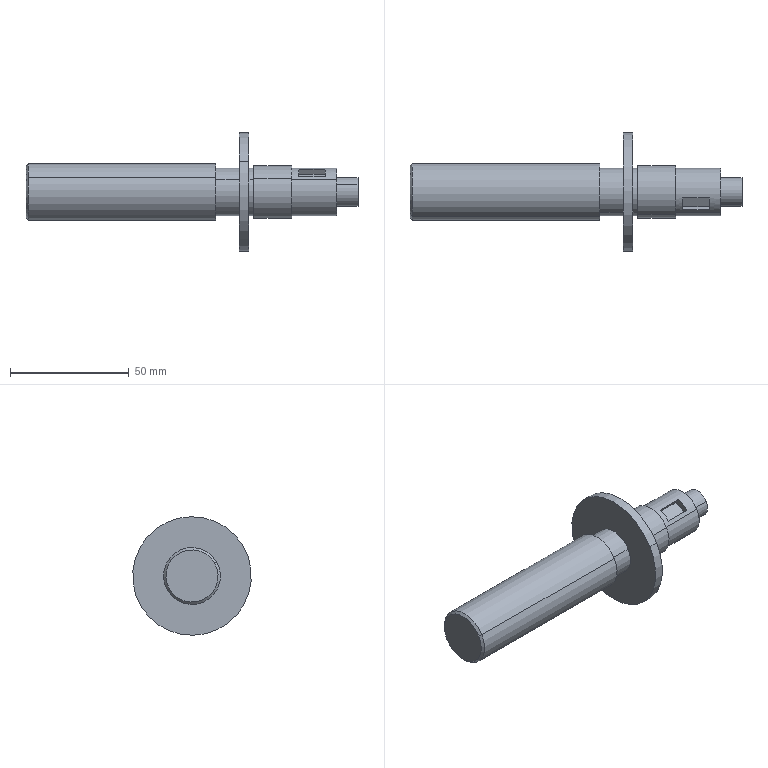Component | SolidWorks | ScrewRod-1 | 1 solid | 29 faces | box 140 x 50 x 50 mm | volume 60656 mm3 | cylinder 14 | plane 13 | cone 2 | commonest cylinder face diameters 20 x6 24 x2 50 x2 22 x2 12 x2
STEP:
#1=COLOUR_RGB('',0.7922,0.8196,0.9333);
#2=FILL_AREA_STYLE_COLOUR('',#1);
#3=FILL_AREA_STYLE('',(#2));
#4=SURFACE_STYLE_FILL_AREA(#3);
#5=SURFACE_SIDE_STYLE('',(#4));
#6=SURFACE_STYLE_USAGE(.BOTH.,#5);
#7=PRESENTATION_STYLE_ASSIGNMENT((#6));
#8=CARTESIAN_POINT('',(0.7305,6.278,-0.8121));
#9=VERTEX_POINT('',#8);
#10=CARTESIAN_POINT('',(0.7305,5.533,-0.369));
#11=VERTEX_POINT('',#10);
#12=CARTESIAN_POINT('',(0.7305,5.906,-0.5906));
#13=DIRECTION('',(-1.,-0.,0.));
#14=DIRECTION('',(0.,-0.8593,0.5115));
#15=AXIS2_PLACEMENT_3D('',#12,#13,#14);
#16=CIRCLE('',#15,0.4331);
#17=EDGE_CURVE('',#9,#11,#16,.T.);
#18=ORIENTED_EDGE('',*,*,#17,.F.);
#19=CARTESIAN_POINT('',(0.7699,6.311,-0.8322));
#20=VERTEX_POINT('',#19);
#21=CARTESIAN_POINT('',(0.7305,6.278,-0.8121));
#22=DIRECTION('',(0.7071,0.6076,-0.3617));
#23=VECTOR('',#22,39.37);
#24=LINE('',#21,#23);
#25=EDGE_CURVE('',#9,#20,#24,.T.);
#26=ORIENTED_EDGE('',*,*,#25,.T.);
#27=CARTESIAN_POINT('',(0.7699,5.5,-0.3489));
#28=VERTEX_POINT('',#27);
#29=CARTESIAN_POINT('',(0.7699,5.906,-0.5906));
#30=DIRECTION('',(1.,0.,-0.));
#31=DIRECTION('',(0.,-0.8593,0.5115));
#32=AXIS2_PLACEMENT_3D('',#29,#30,#31);
#33=CIRCLE('',#32,0.4724);
#34=EDGE_CURVE('',#28,#20,#33,.T.);
#35=ORIENTED_EDGE('',*,*,#34,.F.);
#36=CARTESIAN_POINT('',(0.7305,5.533,-0.369));
#37=DIRECTION('',(0.7071,-0.6076,0.3617));
#38=VECTOR('',#37,39.37);
#39=LINE('',#36,#38);
#40=EDGE_CURVE('',#11,#28,#39,.T.);
#41=ORIENTED_EDGE('',*,*,#40,.F.);
#42=EDGE_LOOP('',(#18,#26,#35,#41));
#43=FACE_OUTER_BOUND('',#42,.T.);
#44=CARTESIAN_POINT('',(0.7305,5.906,-0.5906));
#45=DIRECTION('',(1.,0.,-0.));
#46=DIRECTION('',(0.,-0.8593,0.5115));
#47=AXIS2_PLACEMENT_3D('',#44,#45,#46);
#48=CONICAL_SURFACE('',#47,0.4331,0.7854);
#49=ADVANCED_FACE('',(#43),#48,.T.);
#50=CARTESIAN_POINT('',(3.88,6.311,-0.8322));
#51=VERTEX_POINT('',#50);
#52=CARTESIAN_POINT('',(3.88,5.5,-0.3489));
#53=VERTEX_POINT('',#52);
#54=CARTESIAN_POINT('',(3.88,5.906,-0.5906));
#55=DIRECTION('',(-1.,-0.,0.));
#56=DIRECTION('',(0.,0.8593,-0.5115));
#57=AXIS2_PLACEMENT_3D('',#54,#55,#56);
#58=CIRCLE('',#57,0.4724);
#59=EDGE_CURVE('',#51,#53,#58,.T.);
#60=ORIENTED_EDGE('',*,*,#59,.T.);
#61=CARTESIAN_POINT('',(0.7305,5.5,-0.3489));
#62=DIRECTION('',(-1.,-0.,0.));
#63=VECTOR('',#62,39.37);
#64=LINE('',#61,#63);
#65=EDGE_CURVE('',#53,#28,#64,.T.);
#66=ORIENTED_EDGE('',*,*,#65,.T.);
#67=ORIENTED_EDGE('',*,*,#34,.T.);
#68=CARTESIAN_POINT('',(0.7305,6.311,-0.8322));
#69=DIRECTION('',(-1.,-0.,0.));
#70=VECTOR('',#69,39.37);
#71=LINE('',#68,#70);
#72=EDGE_CURVE('',#51,#20,#71,.T.);
#73=ORIENTED_EDGE('',*,*,#72,.F.);
#74=EDGE_LOOP('',(#60,#66,#67,#73));
#75=FACE_OUTER_BOUND('',#74,.T.);
#76=CARTESIAN_POINT('',(0.7305,5.906,-0.5906));
#77=DIRECTION('',(-1.,-0.,0.));
#78=DIRECTION('',(0.,0.8593,-0.5115));
#79=AXIS2_PLACEMENT_3D('',#76,#77,#78);
#80=CYLINDRICAL_SURFACE('',#79,0.4724);
#81=ADVANCED_FACE('',(#75),#80,.T.);
#82=CARTESIAN_POINT('',(4.274,6.244,-0.7919));
#83=VERTEX_POINT('',#82);
#84=CARTESIAN_POINT('',(4.274,5.567,-0.3892));
#85=VERTEX_POINT('',#84);
#86=CARTESIAN_POINT('',(4.274,5.906,-0.5906));
#87=DIRECTION('',(-1.,-0.,0.));
#88=DIRECTION('',(0.,0.8593,-0.5115));
#89=AXIS2_PLACEMENT_3D('',#86,#87,#88);
#90=CIRCLE('',#89,0.3937);
#91=EDGE_CURVE('',#83,#85,#90,.T.);
#92=ORIENTED_EDGE('',*,*,#91,.T.);
#93=CARTESIAN_POINT('',(3.88,5.567,-0.3892));
#94=VERTEX_POINT('',#93);
#95=CARTESIAN_POINT('',(0.7305,5.567,-0.3892));
#96=DIRECTION('',(-1.,-0.,0.));
#97=VECTOR('',#96,39.37);
#98=LINE('',#95,#97);
#99=EDGE_CURVE('',#85,#94,#98,.T.);
#100=ORIENTED_EDGE('',*,*,#99,.T.);
#101=CARTESIAN_POINT('',(3.88,6.244,-0.7919));
#102=VERTEX_POINT('',#101);
#103=CARTESIAN_POINT('',(3.88,5.906,-0.5906));
#104=DIRECTION('',(-1.,-0.,0.));
#105=DIRECTION('',(0.,0.8593,-0.5115));
#106=AXIS2_PLACEMENT_3D('',#103,#104,#105);
#107=CIRCLE('',#106,0.3937);
#108=EDGE_CURVE('',#102,#94,#107,.T.);
#109=ORIENTED_EDGE('',*,*,#108,.F.);
#110=CARTESIAN_POINT('',(0.7305,6.244,-0.7919));
#111=DIRECTION('',(-1.,-0.,0.));
#112=VECTOR('',#111,39.37);
#113=LINE('',#110,#112);
#114=EDGE_CURVE('',#83,#102,#113,.T.);
#115=ORIENTED_EDGE('',*,*,#114,.F.);
#116=EDGE_LOOP('',(#92,#100,#109,#115));
#117=FACE_OUTER_BOUND('',#116,.T.);
#118=CARTESIAN_POINT('',(0.7305,5.906,-0.5906));
#119=DIRECTION('',(-1.,-0.,0.));
#120=DIRECTION('',(0.,0.8593,-0.5115));
#121=AXIS2_PLACEMENT_3D('',#118,#119,#120);
#122=CYLINDRICAL_SURFACE('',#121,0.3937);
#123=ADVANCED_FACE('',(#117),#122,.T.);
#124=CARTESIAN_POINT('',(4.431,6.751,-1.094));
#125=VERTEX_POINT('',#124);
#126=CARTESIAN_POINT('',(4.431,5.06,-0.08708));
#127=VERTEX_POINT('',#126);
#128=CARTESIAN_POINT('',(4.431,5.906,-0.5906));
#129=DIRECTION('',(-1.,-0.,0.));
#130=DIRECTION('',(0.,0.8593,-0.5115));
#131=AXIS2_PLACEMENT_3D('',#128,#129,#130);
#132=CIRCLE('',#131,0.9843);
#133=EDGE_CURVE('',#125,#127,#132,.T.);
#134=ORIENTED_EDGE('',*,*,#133,.T.);
#135=CARTESIAN_POINT('',(4.274,5.06,-0.08708));
#136=VERTEX_POINT('',#135);
#137=CARTESIAN_POINT('',(0.7305,5.06,-0.08708));
#138=DIRECTION('',(-1.,-0.,0.));
#139=VECTOR('',#138,39.37);
#140=LINE('',#137,#139);
#141=EDGE_CURVE('',#127,#136,#140,.T.);
#142=ORIENTED_EDGE('',*,*,#141,.T.);
#143=CARTESIAN_POINT('',(4.274,6.751,-1.094));
#144=VERTEX_POINT('',#143);
#145=CARTESIAN_POINT('',(4.274,5.906,-0.5906));
#146=DIRECTION('',(-1.,-0.,0.));
#147=DIRECTION('',(0.,0.8593,-0.5115));
#148=AXIS2_PLACEMENT_3D('',#145,#146,#147);
#149=CIRCLE('',#148,0.9843);
#150=EDGE_CURVE('',#144,#136,#149,.T.);
#151=ORIENTED_EDGE('',*,*,#150,.F.);
#152=CARTESIAN_POINT('',(0.7305,6.751,-1.094));
#153=DIRECTION('',(-1.,-0.,0.));
#154=VECTOR('',#153,39.37);
#155=LINE('',#152,#154);
#156=EDGE_CURVE('',#125,#144,#155,.T.);
#157=ORIENTED_EDGE('',*,*,#156,.F.);
#158=EDGE_LOOP('',(#134,#142,#151,#157));
#159=FACE_OUTER_BOUND('',#158,.T.);
#160=CARTESIAN_POINT('',(0.7305,5.906,-0.5906));
#161=DIRECTION('',(-1.,-0.,0.));
#162=DIRECTION('',(-0.,0.8593,-0.5115));
#163=AXIS2_PLACEMENT_3D('',#160,#161,#162);
#164=CYLINDRICAL_SURFACE('',#163,0.9843);
#165=ADVANCED_FACE('',(#159),#164,.T.);
#166=CARTESIAN_POINT('',(4.51,6.244,-0.7919));
#167=VERTEX_POINT('',#166);
#168=CARTESIAN_POINT('',(4.51,5.567,-0.3892));
#169=VERTEX_POINT('',#168);
#170=CARTESIAN_POINT('',(4.51,5.906,-0.5906));
#171=DIRECTION('',(-1.,-0.,0.));
#172=DIRECTION('',(0.,0.8593,-0.5115));
#173=AXIS2_PLACEMENT_3D('',#170,#171,#172);
#174=CIRCLE('',#173,0.3937);
#175=EDGE_CURVE('',#167,#169,#174,.T.);
#176=ORIENTED_EDGE('',*,*,#175,.T.);
#177=CARTESIAN_POINT('',(4.431,5.567,-0.3892));
#178=VERTEX_POINT('',#177);
#179=CARTESIAN_POINT('',(0.7305,5.567,-0.3892));
#180=DIRECTION('',(-1.,-0.,0.));
#181=VECTOR('',#180,39.37);
#182=LINE('',#179,#181);
#183=EDGE_CURVE('',#169,#178,#182,.T.);
#184=ORIENTED_EDGE('',*,*,#183,.T.);
#185=CARTESIAN_POINT('',(4.431,6.244,-0.7919));
#186=VERTEX_POINT('',#185);
#187=CARTESIAN_POINT('',(4.431,5.906,-0.5906));
#188=DIRECTION('',(-1.,-0.,0.));
#189=DIRECTION('',(0.,0.8593,-0.5115));
#190=AXIS2_PLACEMENT_3D('',#187,#188,#189);
#191=CIRCLE('',#190,0.3937);
#192=EDGE_CURVE('',#186,#178,#191,.T.);
#193=ORIENTED_EDGE('',*,*,#192,.F.);
#194=CARTESIAN_POINT('',(0.7305,6.244,-0.7919));
#195=DIRECTION('',(-1.,-0.,0.));
#196=VECTOR('',#195,39.37);
#197=LINE('',#194,#196);
#198=EDGE_CURVE('',#167,#186,#197,.T.);
#199=ORIENTED_EDGE('',*,*,#198,.F.);
#200=EDGE_LOOP('',(#176,#184,#193,#199));
#201=FACE_OUTER_BOUND('',#200,.T.);
#202=CARTESIAN_POINT('',(0.7305,5.906,-0.5906));
#203=DIRECTION('',(-1.,-0.,0.));
#204=DIRECTION('',(0.,0.8593,-0.5115));
#205=AXIS2_PLACEMENT_3D('',#202,#203,#204);
#206=CYLINDRICAL_SURFACE('',#205,0.3937);
#207=ADVANCED_FACE('',(#201),#206,.T.);
#208=CARTESIAN_POINT('',(5.14,6.278,-0.8121));
#209=VERTEX_POINT('',#208);
#210=CARTESIAN_POINT('',(5.14,5.533,-0.369));
#211=VERTEX_POINT('',#210);
#212=CARTESIAN_POINT('',(5.14,5.906,-0.5906));
#213=DIRECTION('',(-1.,-0.,0.));
#214=DIRECTION('',(0.,0.8593,-0.5115));
#215=AXIS2_PLACEMENT_3D('',#212,#213,#214);
#216=CIRCLE('',#215,0.4331);
#217=EDGE_CURVE('',#209,#211,#216,.T.);
#218=ORIENTED_EDGE('',*,*,#217,.T.);
#219=CARTESIAN_POINT('',(4.51,5.533,-0.369));
#220=VERTEX_POINT('',#219);
#221=CARTESIAN_POINT('',(0.7305,5.533,-0.369));
#222=DIRECTION('',(-1.,-0.,0.));
#223=VECTOR('',#222,39.37);
#224=LINE('',#221,#223);
#225=EDGE_CURVE('',#211,#220,#224,.T.);
#226=ORIENTED_EDGE('',*,*,#225,.T.);
#227=CARTESIAN_POINT('',(4.51,6.278,-0.8121));
#228=VERTEX_POINT('',#227);
#229=CARTESIAN_POINT('',(4.51,5.906,-0.5906));
#230=DIRECTION('',(-1.,-0.,0.));
#231=DIRECTION('',(0.,0.8593,-0.5115));
#232=AXIS2_PLACEMENT_3D('',#229,#230,#231);
#233=CIRCLE('',#232,0.4331);
#234=EDGE_CURVE('',#228,#220,#233,.T.);
#235=ORIENTED_EDGE('',*,*,#234,.F.);
#236=CARTESIAN_POINT('',(0.7305,6.278,-0.8121));
#237=DIRECTION('',(-1.,-0.,0.));
#238=VECTOR('',#237,39.37);
#239=LINE('',#236,#238);
#240=EDGE_CURVE('',#209,#228,#239,.T.);
#241=ORIENTED_EDGE('',*,*,#240,.F.);
#242=EDGE_LOOP('',(#218,#226,#235,#241));
#243=FACE_OUTER_BOUND('',#242,.T.);
#244=CARTESIAN_POINT('',(0.7305,5.906,-0.5906));
#245=DIRECTION('',(-1.,-0.,0.));
#246=DIRECTION('',(0.,0.8593,-0.5115));
#247=AXIS2_PLACEMENT_3D('',#244,#245,#246);
#248=CYLINDRICAL_SURFACE('',#247,0.4331);
#249=ADVANCED_FACE('',(#243),#248,.T.);
#250=CARTESIAN_POINT('',(6.242,6.108,-0.7114));
#251=VERTEX_POINT('',#250);
#252=CARTESIAN_POINT('',(6.242,5.703,-0.4697));
#253=VERTEX_POINT('',#252);
#254=CARTESIAN_POINT('',(6.242,5.906,-0.5906));
#255=DIRECTION('',(-1.,-0.,0.));
#256=DIRECTION('',(0.,0.8593,-0.5115));
#257=AXIS2_PLACEMENT_3D('',#254,#255,#256);
#258=CIRCLE('',#257,0.2362);
#259=EDGE_CURVE('',#251,#253,#258,.T.);
#260=ORIENTED_EDGE('',*,*,#259,.T.);
#261=CARTESIAN_POINT('',(5.888,5.703,-0.4697));
#262=VERTEX_POINT('',#261);
#263=CARTESIAN_POINT('',(0.7305,5.703,-0.4697));
#264=DIRECTION('',(-1.,-0.,0.));
#265=VECTOR('',#264,39.37);
#266=LINE('',#263,#265);
#267=EDGE_CURVE('',#253,#262,#266,.T.);
#268=ORIENTED_EDGE('',*,*,#267,.T.);
#269=CARTESIAN_POINT('',(5.888,6.108,-0.7114));
#270=VERTEX_POINT('',#269);
#271=CARTESIAN_POINT('',(5.888,5.906,-0.5906));
#272=DIRECTION('',(-1.,-0.,0.));
#273=DIRECTION('',(0.,0.8593,-0.5115));
#274=AXIS2_PLACEMENT_3D('',#271,#272,#273);
#275=CIRCLE('',#274,0.2362);
#276=EDGE_CURVE('',#270,#262,#275,.T.);
#277=ORIENTED_EDGE('',*,*,#276,.F.);
#278=CARTESIAN_POINT('',(0.7305,6.108,-0.7114));
#279=DIRECTION('',(-1.,-0.,0.));
#280=VECTOR('',#279,39.37);
#281=LINE('',#278,#280);
#282=EDGE_CURVE('',#251,#270,#281,.T.);
#283=ORIENTED_EDGE('',*,*,#282,.F.);
#284=EDGE_LOOP('',(#260,#268,#277,#283));
#285=FACE_OUTER_BOUND('',#284,.T.);
#286=CARTESIAN_POINT('',(0.7305,5.906,-0.5906));
#287=DIRECTION('',(-1.,-0.,0.));
#288=DIRECTION('',(0.,0.8593,-0.5115));
#289=AXIS2_PLACEMENT_3D('',#286,#287,#288);
#290=CYLINDRICAL_SURFACE('',#289,0.2362);
#291=ADVANCED_FACE('',(#285),#290,.T.);
#292=CARTESIAN_POINT('',(5.888,6.244,-0.7919));
#293=VERTEX_POINT('',#292);
#294=CARTESIAN_POINT('',(5.888,5.567,-0.3892));
#295=VERTEX_POINT('',#294);
#296=CARTESIAN_POINT('',(5.888,5.906,-0.5906));
#297=DIRECTION('',(-1.,-0.,0.));
#298=DIRECTION('',(0.,0.8593,-0.5115));
#299=AXIS2_PLACEMENT_3D('',#296,#297,#298);
#300=CIRCLE('',#299,0.3937);
#301=EDGE_CURVE('',#293,#295,#300,.T.);
#302=ORIENTED_EDGE('',*,*,#301,.T.);
#303=CARTESIAN_POINT('',(5.14,5.567,-0.3892));
#304=VERTEX_POINT('',#303);
#305=CARTESIAN_POINT('',(0.7305,5.567,-0.3892));
#306=DIRECTION('',(-1.,-0.,0.));
#307=VECTOR('',#306,39.37);
#308=LINE('',#305,#307);
#309=EDGE_CURVE('',#295,#304,#308,.T.);
#310=ORIENTED_EDGE('',*,*,#309,.T.);
#311=CARTESIAN_POINT('',(5.14,6.244,-0.7919));
#312=VERTEX_POINT('',#311);
#313=CARTESIAN_POINT('',(5.14,5.906,-0.5906));
#314=DIRECTION('',(-1.,-0.,0.));
#315=DIRECTION('',(0.,0.8593,-0.5115));
#316=AXIS2_PLACEMENT_3D('',#313,#314,#315);
#317=CIRCLE('',#316,0.3937);
#318=EDGE_CURVE('',#312,#304,#317,.T.);
#319=ORIENTED_EDGE('',*,*,#318,.F.);
#320=CARTESIAN_POINT('',(0.7305,6.244,-0.7919));
#321=DIRECTION('',(-1.,-0.,0.));
#322=VECTOR('',#321,39.37);
#323=LINE('',#320,#322);
#324=EDGE_CURVE('',#293,#312,#323,.T.);
#325=ORIENTED_EDGE('',*,*,#324,.F.);
#326=EDGE_LOOP('',(#302,#310,#319,#325));
#327=FACE_OUTER_BOUND('',#326,.T.);
#328=CARTESIAN_POINT('',(0.7305,5.906,-0.5906));
#329=DIRECTION('',(-1.,-0.,0.));
#330=DIRECTION('',(0.,0.8593,-0.5115));
#331=AXIS2_PLACEMENT_3D('',#328,#329,#330);
#332=CYLINDRICAL_SURFACE('',#331,0.3937);
#333=ADVANCED_FACE('',(#327),#332,.T.);
#334=ORIENTED_EDGE('',*,*,#309,.F.);
#335=CARTESIAN_POINT('',(5.888,5.906,-0.5906));
#336=DIRECTION('',(-1.,-0.,0.));
#337=DIRECTION('',(0.,0.8593,-0.5115));
#338=AXIS2_PLACEMENT_3D('',#335,#336,#337);
#339=CIRCLE('',#338,0.3937);
#340=EDGE_CURVE('',#295,#293,#339,.T.);
#341=ORIENTED_EDGE('',*,*,#340,.T.);
#342=ORIENTED_EDGE('',*,*,#324,.T.);
#343=CARTESIAN_POINT('',(5.14,5.906,-0.5906));
#344=DIRECTION('',(-1.,-0.,0.));
#345=DIRECTION('',(0.,0.8593,-0.5115));
#346=AXIS2_PLACEMENT_3D('',#343,#344,#345);
#347=CIRCLE('',#346,0.3937);
#348=EDGE_CURVE('',#304,#312,#347,.T.);
#349=ORIENTED_EDGE('',*,*,#348,.F.);
#350=EDGE_LOOP('',(#334,#341,#342,#349));
#351=FACE_OUTER_BOUND('',#350,.T.);
#352=CARTESIAN_POINT('',(5.262,5.807,-0.2094));
#353=VERTEX_POINT('',#352);
#354=CARTESIAN_POINT('',(5.262,5.606,-0.3345));
#355=VERTEX_POINT('',#354);
#356=CARTESIAN_POINT('',(5.262,5.906,-0.5906));
#357=DIRECTION('',(1.,0.,-0.));
#358=DIRECTION('',(0.,-0.8593,0.5115));
#359=AXIS2_PLACEMENT_3D('',#356,#357,#358);
#360=CIRCLE('',#359,0.3937);
#361=EDGE_CURVE('',#353,#355,#360,.T.);
#362=ORIENTED_EDGE('',*,*,#361,.F.);
#363=CARTESIAN_POINT('',(5.695,5.807,-0.2094));
#364=VERTEX_POINT('',#363);
#365=CARTESIAN_POINT('',(5.262,5.807,-0.2094));
#366=DIRECTION('',(1.,0.,-0.));
#367=VECTOR('',#366,39.37);
#368=LINE('',#365,#367);
#369=EDGE_CURVE('',#353,#364,#368,.T.);
#370=ORIENTED_EDGE('',*,*,#369,.T.);
#371=CARTESIAN_POINT('',(5.695,5.606,-0.3345));
#372=VERTEX_POINT('',#371);
#373=CARTESIAN_POINT('',(5.695,5.906,-0.5906));
#374=DIRECTION('',(1.,0.,-0.));
#375=DIRECTION('',(0.,-0.8593,0.5115));
#376=AXIS2_PLACEMENT_3D('',#373,#374,#375);
#377=CIRCLE('',#376,0.3937);
#378=EDGE_CURVE('',#364,#372,#377,.T.);
#379=ORIENTED_EDGE('',*,*,#378,.T.);
#380=CARTESIAN_POINT('',(5.262,5.606,-0.3345));
#381=DIRECTION('',(1.,0.,-0.));
#382=VECTOR('',#381,39.37);
#383=LINE('',#380,#382);
#384=EDGE_CURVE('',#355,#372,#383,.T.);
#385=ORIENTED_EDGE('',*,*,#384,.F.);
#386=EDGE_LOOP('',(#362,#370,#379,#385));
#387=FACE_BOUND('',#386,.T.);
#388=CARTESIAN_POINT('',(0.7305,5.906,-0.5906));
#389=DIRECTION('',(-1.,-0.,0.));
#390=DIRECTION('',(0.,0.8593,-0.5115));
#391=AXIS2_PLACEMENT_3D('',#388,#389,#390);
#392=CYLINDRICAL_SURFACE('',#391,0.3937);
#393=ADVANCED_FACE('',(#351,#387),#392,.T.);
#394=ORIENTED_EDGE('',*,*,#259,.F.);
#395=CARTESIAN_POINT('',(6.242,5.906,-0.5906));
#396=DIRECTION('',(-1.,-0.,0.));
#397=DIRECTION('',(0.,0.8593,-0.5115));
#398=AXIS2_PLACEMENT_3D('',#395,#396,#397);
#399=CIRCLE('',#398,0.2362);
#400=EDGE_CURVE('',#253,#251,#399,.T.);
#401=ORIENTED_EDGE('',*,*,#400,.F.);
#402=EDGE_LOOP('',(#394,#401));
#403=FACE_OUTER_BOUND('',#402,.T.);
#404=CARTESIAN_POINT('',(6.242,5.906,-0.5906));
#405=DIRECTION('',(-1.,-0.,0.));
#406=DIRECTION('',(-0.,0.8593,-0.5115));
#407=AXIS2_PLACEMENT_3D('',#404,#405,#406);
#408=PLANE('',#407);
#409=ADVANCED_FACE('',(#403),#408,.F.);
#410=ORIENTED_EDGE('',*,*,#267,.F.);
#411=ORIENTED_EDGE('',*,*,#400,.T.);
#412=ORIENTED_EDGE('',*,*,#282,.T.);
#413=CARTESIAN_POINT('',(5.888,5.906,-0.5906));
#414=DIRECTION('',(-1.,-0.,0.));
#415=DIRECTION('',(0.,0.8593,-0.5115));
#416=AXIS2_PLACEMENT_3D('',#413,#414,#415);
#417=CIRCLE('',#416,0.2362);
#418=EDGE_CURVE('',#262,#270,#417,.T.);
#419=ORIENTED_EDGE('',*,*,#418,.F.);
#420=EDGE_LOOP('',(#410,#411,#412,#419));
#421=FACE_OUTER_BOUND('',#420,.T.);
#422=CARTESIAN_POINT('',(0.7305,5.906,-0.5906));
#423=DIRECTION('',(-1.,-0.,0.));
#424=DIRECTION('',(0.,0.8593,-0.5115));
#425=AXIS2_PLACEMENT_3D('',#422,#423,#424);
#426=CYLINDRICAL_SURFACE('',#425,0.2362);
#427=ADVANCED_FACE('',(#421),#426,.T.);
#428=ORIENTED_EDGE('',*,*,#301,.F.);
#429=ORIENTED_EDGE('',*,*,#340,.F.);
#430=EDGE_LOOP('',(#428,#429));
#431=FACE_OUTER_BOUND('',#430,.T.);
#432=ORIENTED_EDGE('',*,*,#276,.T.);
#433=ORIENTED_EDGE('',*,*,#418,.T.);
#434=EDGE_LOOP('',(#432,#433));
#435=FACE_BOUND('',#434,.T.);
#436=CARTESIAN_POINT('',(5.888,5.785,-0.7935));
#437=DIRECTION('',(-1.,-0.,0.));
#438=DIRECTION('',(-0.,0.8593,-0.5115));
#439=AXIS2_PLACEMENT_3D('',#436,#437,#438);
#440=PLANE('',#439);
#441=ADVANCED_FACE('',(#431,#435),#440,.F.);
#442=ORIENTED_EDGE('',*,*,#217,.F.);
#443=CARTESIAN_POINT('',(5.14,5.906,-0.5906));
#444=DIRECTION('',(-1.,-0.,0.));
#445=DIRECTION('',(0.,0.8593,-0.5115));
#446=AXIS2_PLACEMENT_3D('',#443,#444,#445);
#447=CIRCLE('',#446,0.4331);
#448=EDGE_CURVE('',#211,#209,#447,.T.);
#449=ORIENTED_EDGE('',*,*,#448,.F.);
#450=EDGE_LOOP('',(#442,#449));
#451=FACE_OUTER_BOUND('',#450,.T.);
#452=ORIENTED_EDGE('',*,*,#318,.T.);
#453=ORIENTED_EDGE('',*,*,#348,.T.);
#454=EDGE_LOOP('',(#452,#453));
#455=FACE_BOUND('',#454,.T.);
#456=CARTESIAN_POINT('',(5.14,5.684,-0.9627));
#457=DIRECTION('',(-1.,-0.,0.));
#458=DIRECTION('',(-0.,0.8593,-0.5115));
#459=AXIS2_PLACEMENT_3D('',#456,#457,#458);
#460=PLANE('',#459);
#461=ADVANCED_FACE('',(#451,#455),#460,.F.);
#462=ORIENTED_EDGE('',*,*,#225,.F.);
#463=ORIENTED_EDGE('',*,*,#448,.T.);
#464=ORIENTED_EDGE('',*,*,#240,.T.);
#465=CARTESIAN_POINT('',(4.51,5.906,-0.5906));
#466=DIRECTION('',(-1.,-0.,0.));
#467=DIRECTION('',(0.,0.8593,-0.5115));
#468=AXIS2_PLACEMENT_3D('',#465,#466,#467);
#469=CIRCLE('',#468,0.4331);
#470=EDGE_CURVE('',#220,#228,#469,.T.);
#471=ORIENTED_EDGE('',*,*,#470,.F.);
#472=EDGE_LOOP('',(#462,#463,#464,#471));
#473=FACE_OUTER_BOUND('',#472,.T.);
#474=CARTESIAN_POINT('',(0.7305,5.906,-0.5906));
#475=DIRECTION('',(-1.,-0.,0.));
#476=DIRECTION('',(0.,0.8593,-0.5115));
#477=AXIS2_PLACEMENT_3D('',#474,#475,#476);
#478=CYLINDRICAL_SURFACE('',#477,0.4331);
#479=ADVANCED_FACE('',(#473),#478,.T.);
#480=ORIENTED_EDGE('',*,*,#175,.F.);
#481=CARTESIAN_POINT('',(4.51,5.906,-0.5906));
#482=DIRECTION('',(-1.,-0.,0.));
#483=DIRECTION('',(0.,0.8593,-0.5115));
#484=AXIS2_PLACEMENT_3D('',#481,#482,#483);
#485=CIRCLE('',#484,0.3937);
#486=EDGE_CURVE('',#169,#167,#485,.T.);
#487=ORIENTED_EDGE('',*,*,#486,.F.);
#488=EDGE_LOOP('',(#480,#487));
#489=FACE_BOUND('',#488,.T.);
#490=ORIENTED_EDGE('',*,*,#234,.T.);
#491=ORIENTED_EDGE('',*,*,#470,.T.);
#492=EDGE_LOOP('',(#490,#491));
#493=FACE_OUTER_BOUND('',#492,.T.);
#494=CARTESIAN_POINT('',(4.51,5.704,-0.9288));
#495=DIRECTION('',(1.,0.,-0.));
#496=DIRECTION('',(0.,-0.8593,0.5115));
#497=AXIS2_PLACEMENT_3D('',#494,#495,#496);
#498=PLANE('',#497);
#499=ADVANCED_FACE('',(#489,#493),#498,.F.);
#500=ORIENTED_EDGE('',*,*,#183,.F.);
#501=ORIENTED_EDGE('',*,*,#486,.T.);
#502=ORIENTED_EDGE('',*,*,#198,.T.);
#503=CARTESIAN_POINT('',(4.431,5.906,-0.5906));
#504=DIRECTION('',(-1.,-0.,0.));
#505=DIRECTION('',(0.,0.8593,-0.5115));
#506=AXIS2_PLACEMENT_3D('',#503,#504,#505);
#507=CIRCLE('',#506,0.3937);
#508=EDGE_CURVE('',#178,#186,#507,.T.);
#509=ORIENTED_EDGE('',*,*,#508,.F.);
#510=EDGE_LOOP('',(#500,#501,#502,#509));
#511=FACE_OUTER_BOUND('',#510,.T.);
#512=CARTESIAN_POINT('',(0.7305,5.906,-0.5906));
#513=DIRECTION('',(-1.,-0.,0.));
#514=DIRECTION('',(0.,0.8593,-0.5115));
#515=AXIS2_PLACEMENT_3D('',#512,#513,#514);
#516=CYLINDRICAL_SURFACE('',#515,0.3937);
#517=ADVANCED_FACE('',(#511),#516,.T.);
#518=ORIENTED_EDGE('',*,*,#133,.F.);
#519=CARTESIAN_POINT('',(4.431,5.906,-0.5906));
#520=DIRECTION('',(-1.,-0.,0.));
#521=DIRECTION('',(0.,0.8593,-0.5115));
#522=AXIS2_PLACEMENT_3D('',#519,#520,#521);
#523=CIRCLE('',#522,0.9843);
#524=EDGE_CURVE('',#127,#125,#523,.T.);
#525=ORIENTED_EDGE('',*,*,#524,.F.);
#526=EDGE_LOOP('',(#518,#525));
#527=FACE_OUTER_BOUND('',#526,.T.);
#528=ORIENTED_EDGE('',*,*,#192,.T.);
#529=ORIENTED_EDGE('',*,*,#508,.T.);
#530=EDGE_LOOP('',(#528,#529));
#531=FACE_BOUND('',#530,.T.);
#532=CARTESIAN_POINT('',(4.431,5.402,-1.436));
#533=DIRECTION('',(-1.,-0.,0.));
#534=DIRECTION('',(-0.,0.8593,-0.5115));
#535=AXIS2_PLACEMENT_3D('',#532,#533,#534);
#536=PLANE('',#535);
#537=ADVANCED_FACE('',(#527,#531),#536,.F.);
#538=ORIENTED_EDGE('',*,*,#141,.F.);
#539=ORIENTED_EDGE('',*,*,#524,.T.);
#540=ORIENTED_EDGE('',*,*,#156,.T.);
#541=CARTESIAN_POINT('',(4.274,5.906,-0.5906));
#542=DIRECTION('',(-1.,-0.,0.));
#543=DIRECTION('',(0.,0.8593,-0.5115));
#544=AXIS2_PLACEMENT_3D('',#541,#542,#543);
#545=CIRCLE('',#544,0.9843);
#546=EDGE_CURVE('',#136,#144,#545,.T.);
#547=ORIENTED_EDGE('',*,*,#546,.F.);
#548=EDGE_LOOP('',(#538,#539,#540,#547));
#549=FACE_OUTER_BOUND('',#548,.T.);
#550=CARTESIAN_POINT('',(0.7305,5.906,-0.5906));
#551=DIRECTION('',(-1.,-0.,0.));
#552=DIRECTION('',(-0.,0.8593,-0.5115));
#553=AXIS2_PLACEMENT_3D('',#550,#551,#552);
#554=CYLINDRICAL_SURFACE('',#553,0.9843);
#555=ADVANCED_FACE('',(#549),#554,.T.);
#556=ORIENTED_EDGE('',*,*,#91,.F.);
#557=CARTESIAN_POINT('',(4.274,5.906,-0.5906));
#558=DIRECTION('',(-1.,-0.,0.));
#559=DIRECTION('',(0.,0.8593,-0.5115));
#560=AXIS2_PLACEMENT_3D('',#557,#558,#559);
#561=CIRCLE('',#560,0.3937);
#562=EDGE_CURVE('',#85,#83,#561,.T.);
#563=ORIENTED_EDGE('',*,*,#562,.F.);
#564=EDGE_LOOP('',(#556,#563));
#565=FACE_BOUND('',#564,.T.);
#566=ORIENTED_EDGE('',*,*,#150,.T.);
#567=ORIENTED_EDGE('',*,*,#546,.T.);
#568=EDGE_LOOP('',(#566,#567));
#569=FACE_OUTER_BOUND('',#568,.T.);
#570=CARTESIAN_POINT('',(4.274,5.704,-0.9288));
#571=DIRECTION('',(1.,0.,-0.));
#572=DIRECTION('',(0.,-0.8593,0.5115));
#573=AXIS2_PLACEMENT_3D('',#570,#571,#572);
#574=PLANE('',#573);
#575=ADVANCED_FACE('',(#565,#569),#574,.F.);
#576=ORIENTED_EDGE('',*,*,#99,.F.);
#577=ORIENTED_EDGE('',*,*,#562,.T.);
#578=ORIENTED_EDGE('',*,*,#114,.T.);
#579=CARTESIAN_POINT('',(3.88,5.906,-0.5906));
#580=DIRECTION('',(-1.,-0.,0.));
#581=DIRECTION('',(0.,0.8593,-0.5115));
#582=AXIS2_PLACEMENT_3D('',#579,#580,#581);
#583=CIRCLE('',#582,0.3937);
#584=EDGE_CURVE('',#94,#102,#583,.T.);
#585=ORIENTED_EDGE('',*,*,#584,.F.);
#586=EDGE_LOOP('',(#576,#577,#578,#585));
#587=FACE_OUTER_BOUND('',#586,.T.);
#588=CARTESIAN_POINT('',(0.7305,5.906,-0.5906));
#589=DIRECTION('',(-1.,-0.,0.));
#590=DIRECTION('',(0.,0.8593,-0.5115));
#591=AXIS2_PLACEMENT_3D('',#588,#589,#590);
#592=CYLINDRICAL_SURFACE('',#591,0.3937);
#593=ADVANCED_FACE('',(#587),#592,.T.);
#594=ORIENTED_EDGE('',*,*,#59,.F.);
#595=CARTESIAN_POINT('',(3.88,5.906,-0.5906));
#596=DIRECTION('',(-1.,-0.,0.));
#597=DIRECTION('',(0.,0.8593,-0.5115));
#598=AXIS2_PLACEMENT_3D('',#595,#596,#597);
#599=CIRCLE('',#598,0.4724);
#600=EDGE_CURVE('',#53,#51,#599,.T.);
#601=ORIENTED_EDGE('',*,*,#600,.F.);
#602=EDGE_LOOP('',(#594,#601));
#603=FACE_OUTER_BOUND('',#602,.T.);
#604=ORIENTED_EDGE('',*,*,#108,.T.);
#605=ORIENTED_EDGE('',*,*,#584,.T.);
#606=EDGE_LOOP('',(#604,#605));
#607=FACE_BOUND('',#606,.T.);
#608=CARTESIAN_POINT('',(3.88,5.664,-0.9965));
#609=DIRECTION('',(-1.,-0.,0.));
#610=DIRECTION('',(-0.,0.8593,-0.5115));
#611=AXIS2_PLACEMENT_3D('',#608,#609,#610);
#612=PLANE('',#611);
#613=ADVANCED_FACE('',(#603,#607),#612,.F.);
#614=ORIENTED_EDGE('',*,*,#65,.F.);
#615=ORIENTED_EDGE('',*,*,#600,.T.);
#616=ORIENTED_EDGE('',*,*,#72,.T.);
#617=CARTESIAN_POINT('',(0.7699,5.906,-0.5906));
#618=DIRECTION('',(1.,0.,-0.));
#619=DIRECTION('',(0.,-0.8593,0.5115));
#620=AXIS2_PLACEMENT_3D('',#617,#618,#619);
#621=CIRCLE('',#620,0.4724);
#622=EDGE_CURVE('',#20,#28,#621,.T.);
#623=ORIENTED_EDGE('',*,*,#622,.T.);
#624=EDGE_LOOP('',(#614,#615,#616,#623));
#625=FACE_OUTER_BOUND('',#624,.T.);
#626=CARTESIAN_POINT('',(0.7305,5.906,-0.5906));
#627=DIRECTION('',(-1.,-0.,0.));
#628=DIRECTION('',(0.,0.8593,-0.5115));
#629=AXIS2_PLACEMENT_3D('',#626,#627,#628);
#630=CYLINDRICAL_SURFACE('',#629,0.4724);
#631=ADVANCED_FACE('',(#625),#630,.T.);
#632=CARTESIAN_POINT('',(0.7305,5.906,-0.5906));
#633=DIRECTION('',(-1.,-0.,0.));
#634=DIRECTION('',(0.,-0.8593,0.5115));
#635=AXIS2_PLACEMENT_3D('',#632,#633,#634);
#636=CIRCLE('',#635,0.4331);
#637=EDGE_CURVE('',#11,#9,#636,.T.);
#638=ORIENTED_EDGE('',*,*,#637,.T.);
#639=ORIENTED_EDGE('',*,*,#17,.T.);
#640=EDGE_LOOP('',(#638,#639));
#641=FACE_OUTER_BOUND('',#640,.T.);
#642=CARTESIAN_POINT('',(0.7305,5.906,-0.5906));
#643=DIRECTION('',(1.,0.,-0.));
#644=DIRECTION('',(0.,-0.8593,0.5115));
#645=AXIS2_PLACEMENT_3D('',#642,#643,#644);
#646=PLANE('',#645);
#647=ADVANCED_FACE('',(#641),#646,.F.);
#648=ORIENTED_EDGE('',*,*,#25,.F.);
#649=ORIENTED_EDGE('',*,*,#637,.F.);
#650=ORIENTED_EDGE('',*,*,#40,.T.);
#651=ORIENTED_EDGE('',*,*,#622,.F.);
#652=EDGE_LOOP('',(#648,#649,#650,#651));
#653=FACE_OUTER_BOUND('',#652,.T.);
#654=CARTESIAN_POINT('',(0.7305,5.906,-0.5906));
#655=DIRECTION('',(1.,0.,-0.));
#656=DIRECTION('',(0.,-0.8593,0.5115));
#657=AXIS2_PLACEMENT_3D('',#654,#655,#656);
#658=CONICAL_SURFACE('',#657,0.4331,0.7854);
#659=ADVANCED_FACE('',(#653),#658,.T.);
#660=CARTESIAN_POINT('',(5.695,5.862,-0.2975));
#661=VERTEX_POINT('',#660);
#662=CARTESIAN_POINT('',(5.695,5.659,-0.4193));
#663=VERTEX_POINT('',#662);
#664=CARTESIAN_POINT('',(5.695,5.764,-0.3561));
#665=DIRECTION('',(-0.,-0.8567,-0.5158));
#666=VECTOR('',#665,39.37);
#667=LINE('',#664,#666);
#668=EDGE_CURVE('',#661,#663,#667,.T.);
#669=ORIENTED_EDGE('',*,*,#668,.F.);
#670=CARTESIAN_POINT('',(5.262,5.862,-0.2975));
#671=VERTEX_POINT('',#670);
#672=CARTESIAN_POINT('',(5.262,5.862,-0.2975));
#673=DIRECTION('',(1.,0.,-0.));
#674=VECTOR('',#673,39.37);
#675=LINE('',#672,#674);
#676=EDGE_CURVE('',#671,#661,#675,.T.);
#677=ORIENTED_EDGE('',*,*,#676,.F.);
#678=CARTESIAN_POINT('',(5.262,5.659,-0.4193));
#679=VERTEX_POINT('',#678);
#680=CARTESIAN_POINT('',(5.262,5.764,-0.3561));
#681=DIRECTION('',(-0.,-0.8567,-0.5158));
#682=VECTOR('',#681,39.37);
#683=LINE('',#680,#682);
#684=EDGE_CURVE('',#671,#679,#683,.T.);
#685=ORIENTED_EDGE('',*,*,#684,.T.);
#686=CARTESIAN_POINT('',(5.262,5.659,-0.4193));
#687=DIRECTION('',(1.,0.,-0.));
#688=VECTOR('',#687,39.37);
#689=LINE('',#686,#688);
#690=EDGE_CURVE('',#679,#663,#689,.T.);
#691=ORIENTED_EDGE('',*,*,#690,.T.);
#692=EDGE_LOOP('',(#669,#677,#685,#691));
#693=FACE_OUTER_BOUND('',#692,.T.);
#694=CARTESIAN_POINT('',(5.262,5.764,-0.3561));
#695=DIRECTION('',(0.,-0.5158,0.8567));
#696=DIRECTION('',(-0.,-0.8567,-0.5158));
#697=AXIS2_PLACEMENT_3D('',#694,#695,#696);
#698=PLANE('',#697);
#699=ADVANCED_FACE('',(#693),#698,.T.);
#700=CARTESIAN_POINT('',(5.695,5.805,-0.6531));
#701=DIRECTION('',(0.,-0.5296,0.8482));
#702=VECTOR('',#701,39.37);
#703=LINE('',#700,#702);
#704=EDGE_CURVE('',#663,#372,#703,.T.);
#705=ORIENTED_EDGE('',*,*,#704,.F.);
#706=ORIENTED_EDGE('',*,*,#690,.F.);
#707=CARTESIAN_POINT('',(5.262,5.805,-0.6531));
#708=DIRECTION('',(0.,-0.5296,0.8482));
#709=VECTOR('',#708,39.37);
#710=LINE('',#707,#709);
#711=EDGE_CURVE('',#679,#355,#710,.T.);
#712=ORIENTED_EDGE('',*,*,#711,.T.);
#713=ORIENTED_EDGE('',*,*,#384,.T.);
#714=EDGE_LOOP('',(#705,#706,#712,#713));
#715=FACE_OUTER_BOUND('',#714,.T.);
#716=CARTESIAN_POINT('',(5.262,5.805,-0.6531));
#717=DIRECTION('',(0.,0.8482,0.5296));
#718=DIRECTION('',(0.,-0.5296,0.8482));
#719=AXIS2_PLACEMENT_3D('',#716,#717,#718);
#720=PLANE('',#719);
#721=ADVANCED_FACE('',(#715),#720,.T.);
#722=CARTESIAN_POINT('',(5.695,6.006,-0.528));
#723=DIRECTION('',(0.,-0.5296,0.8482));
#724=VECTOR('',#723,39.37);
#725=LINE('',#722,#724);
#726=EDGE_CURVE('',#661,#364,#725,.T.);
#727=ORIENTED_EDGE('',*,*,#726,.T.);
#728=ORIENTED_EDGE('',*,*,#369,.F.);
#729=CARTESIAN_POINT('',(5.262,6.006,-0.528));
#730=DIRECTION('',(0.,-0.5296,0.8482));
#731=VECTOR('',#730,39.37);
#732=LINE('',#729,#731);
#733=EDGE_CURVE('',#671,#353,#732,.T.);
#734=ORIENTED_EDGE('',*,*,#733,.F.);
#735=ORIENTED_EDGE('',*,*,#676,.T.);
#736=EDGE_LOOP('',(#727,#728,#734,#735));
#737=FACE_OUTER_BOUND('',#736,.T.);
#738=CARTESIAN_POINT('',(5.262,6.006,-0.528));
#739=DIRECTION('',(0.,0.8482,0.5296));
#740=DIRECTION('',(0.,-0.5296,0.8482));
#741=AXIS2_PLACEMENT_3D('',#738,#739,#740);
#742=PLANE('',#741);
#743=ADVANCED_FACE('',(#737),#742,.F.);
#744=ORIENTED_EDGE('',*,*,#684,.F.);
#745=ORIENTED_EDGE('',*,*,#733,.T.);
#746=ORIENTED_EDGE('',*,*,#361,.T.);
#747=ORIENTED_EDGE('',*,*,#711,.F.);
#748=EDGE_LOOP('',(#744,#745,#746,#747));
#749=FACE_OUTER_BOUND('',#748,.T.);
#750=CARTESIAN_POINT('',(5.262,5.906,-0.5906));
#751=DIRECTION('',(1.,0.,-0.));
#752=DIRECTION('',(0.,-0.8593,0.5115));
#753=AXIS2_PLACEMENT_3D('',#750,#751,#752);
#754=PLANE('',#753);
#755=ADVANCED_FACE('',(#749),#754,.T.);
#756=ORIENTED_EDGE('',*,*,#668,.T.);
#757=ORIENTED_EDGE('',*,*,#704,.T.);
#758=ORIENTED_EDGE('',*,*,#378,.F.);
#759=ORIENTED_EDGE('',*,*,#726,.F.);
#760=EDGE_LOOP('',(#756,#757,#758,#759));
#761=FACE_OUTER_BOUND('',#760,.T.);
#762=CARTESIAN_POINT('',(5.695,5.906,-0.5906));
#763=DIRECTION('',(1.,0.,-0.));
#764=DIRECTION('',(0.,-0.8593,0.5115));
#765=AXIS2_PLACEMENT_3D('',#762,#763,#764);
#766=PLANE('',#765);
#767=ADVANCED_FACE('',(#761),#766,.F.);
#768=CLOSED_SHELL('',(#49,#81,#123,#165,#207,#249,#291,#333,#393,#409,#427,#441,#461,#479,#499,#517,#537,#555,#575,#593,#613,#631,#647,#659,#699,#721,#743,#755,#767));
#769=MANIFOLD_SOLID_BREP('',#768);
#770=STYLED_ITEM('',(#7),#769);
#771=PRESENTATION_LAYER_ASSIGNMENT('','',(#770));
#772=(LENGTH_UNIT()NAMED_UNIT(*)SI_UNIT($,.METRE.));
#773=LENGTH_MEASURE_WITH_UNIT(LENGTH_MEASURE(0.0254),#772);
#774=DIMENSIONAL_EXPONENTS(1.,0.,0.,0.,0.,0.,0.);
#775=(CONVERSION_BASED_UNIT('',#773)LENGTH_UNIT()NAMED_UNIT(#774));
#776=UNCERTAINTY_MEASURE_WITH_UNIT(LENGTH_MEASURE(0.00001),#775,'','');
#777=(NAMED_UNIT(*)PLANE_ANGLE_UNIT()SI_UNIT($,.RADIAN.));
#778=(NAMED_UNIT(*)SI_UNIT($,.STERADIAN.)SOLID_ANGLE_UNIT());
#779=(GEOMETRIC_REPRESENTATION_CONTEXT(3)GLOBAL_UNCERTAINTY_ASSIGNED_CONTEXT((#776))GLOBAL_UNIT_ASSIGNED_CONTEXT((#775,#777,#778))REPRESENTATION_CONTEXT('',''));
#780=MECHANICAL_DESIGN_GEOMETRIC_PRESENTATION_REPRESENTATION('',(#770),#779);
#781=CARTESIAN_POINT('',(0.,0.,0.));
#782=DIRECTION('',(0.,0.,1.));
#783=DIRECTION('',(1.,0.,0.));
#784=AXIS2_PLACEMENT_3D('',#781,#782,#783);
#785=(LENGTH_UNIT()NAMED_UNIT(*)SI_UNIT($,.METRE.));
#786=LENGTH_MEASURE_WITH_UNIT(LENGTH_MEASURE(0.0254),#785);
#787=DIMENSIONAL_EXPONENTS(1.,0.,0.,0.,0.,0.,0.);
#788=(CONVERSION_BASED_UNIT('',#786)LENGTH_UNIT()NAMED_UNIT(#787));
#789=UNCERTAINTY_MEASURE_WITH_UNIT(LENGTH_MEASURE(0.00001),#788,'','');
#790=(NAMED_UNIT(*)PLANE_ANGLE_UNIT()SI_UNIT($,.RADIAN.));
#791=(NAMED_UNIT(*)SI_UNIT($,.STERADIAN.)SOLID_ANGLE_UNIT());
#792=(GEOMETRIC_REPRESENTATION_CONTEXT(3)GLOBAL_UNCERTAINTY_ASSIGNED_CONTEXT((#789))GLOBAL_UNIT_ASSIGNED_CONTEXT((#788,#790,#791))REPRESENTATION_CONTEXT('',''));
#793=ADVANCED_BREP_SHAPE_REPRESENTATION('',(#769,#784),#792);